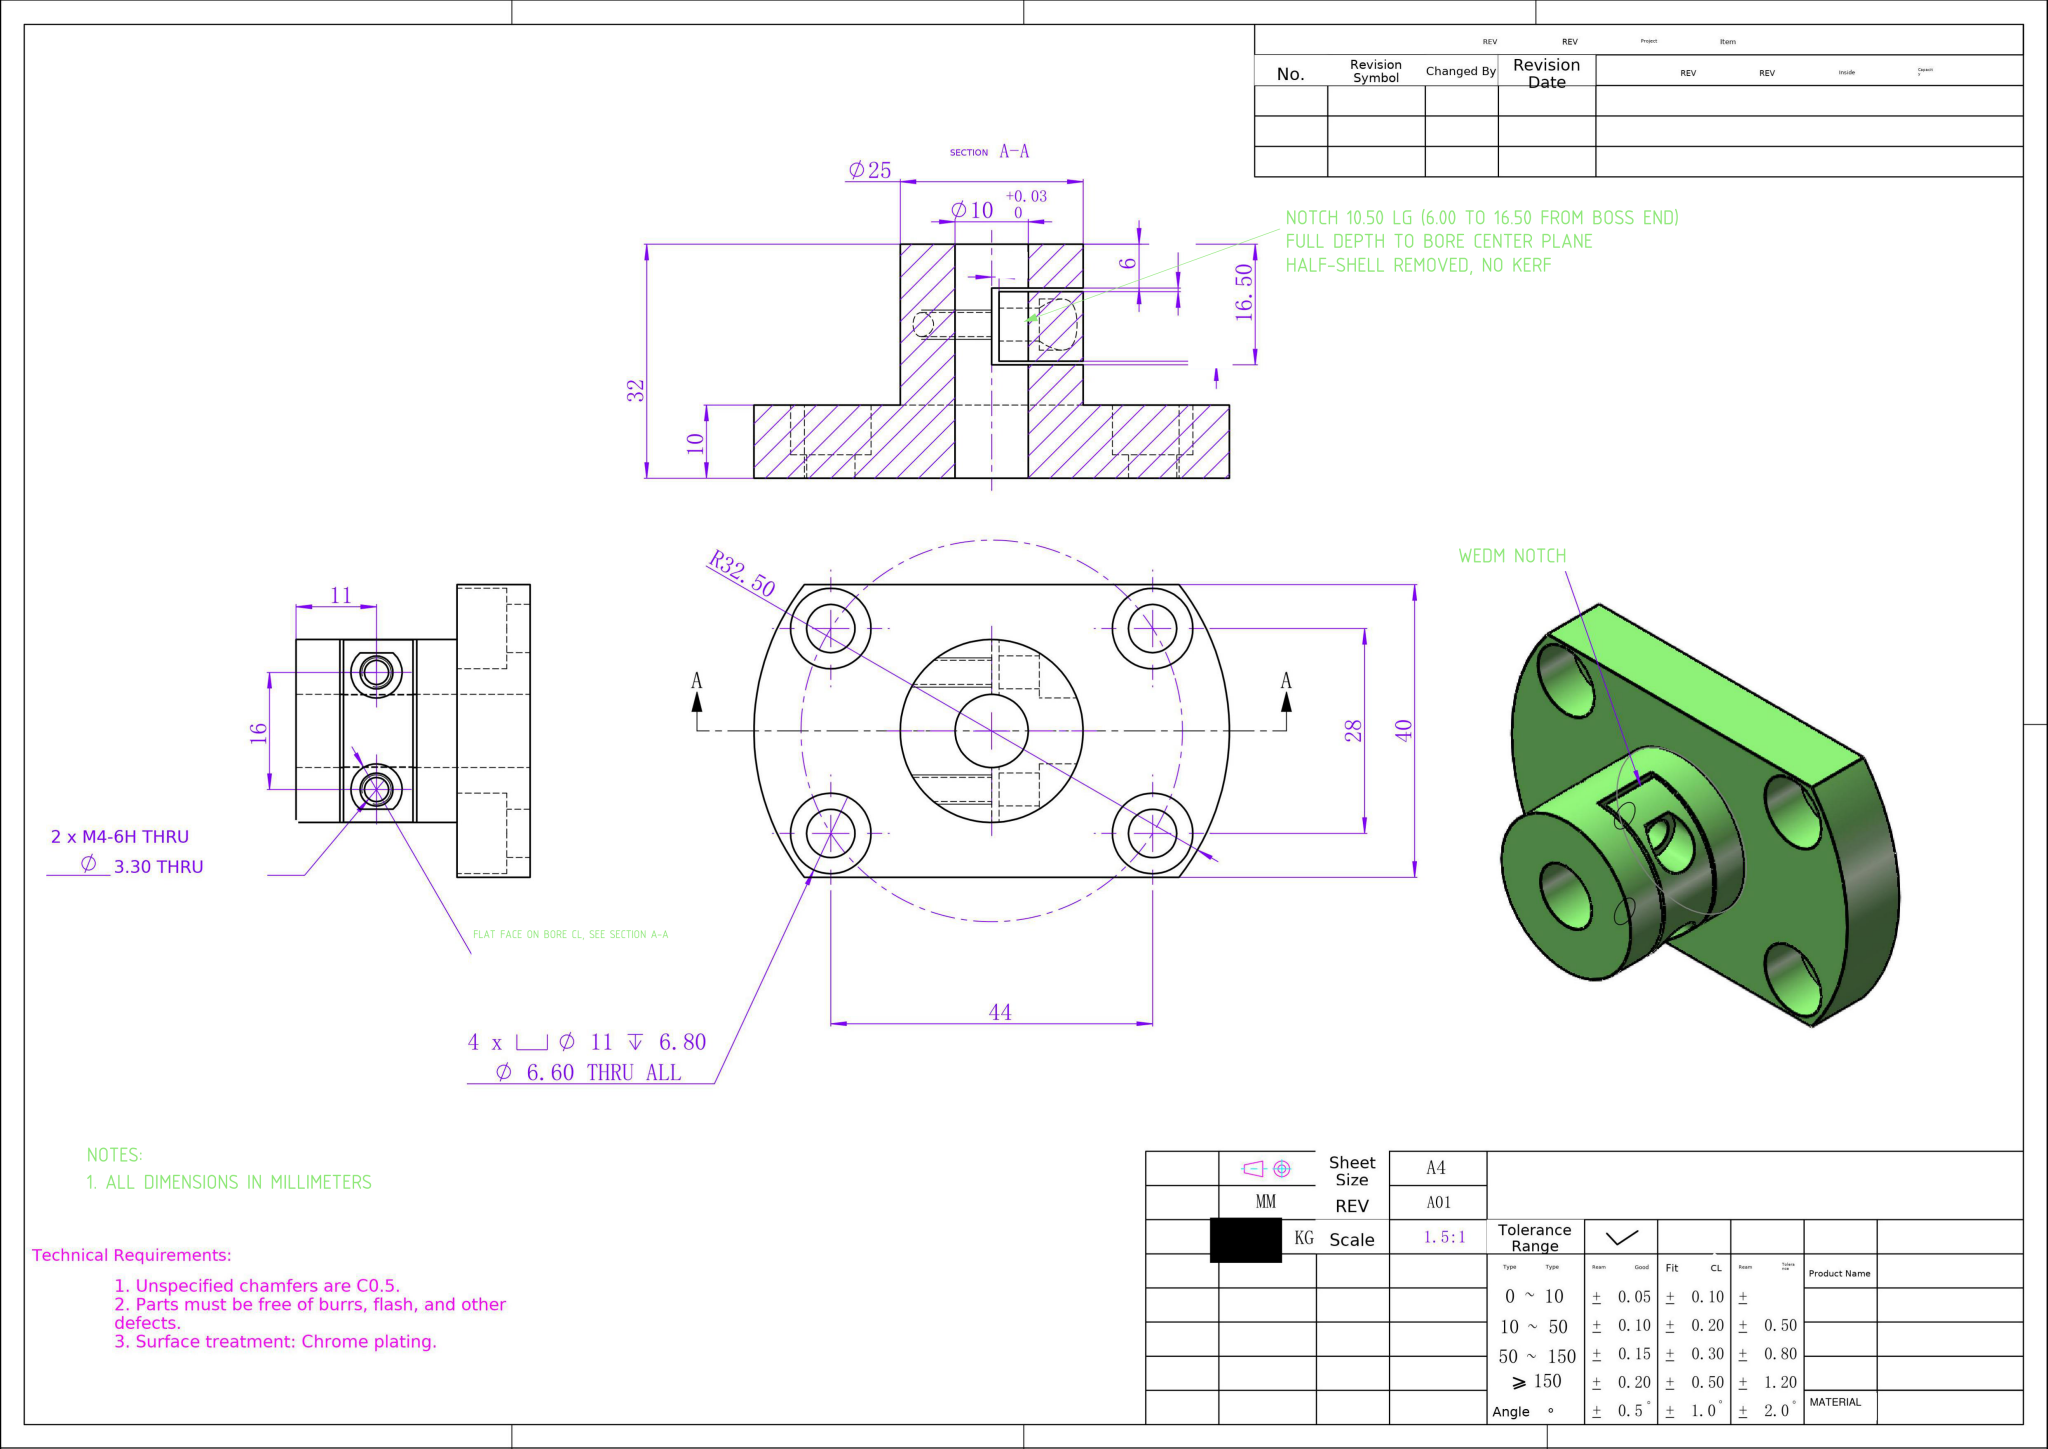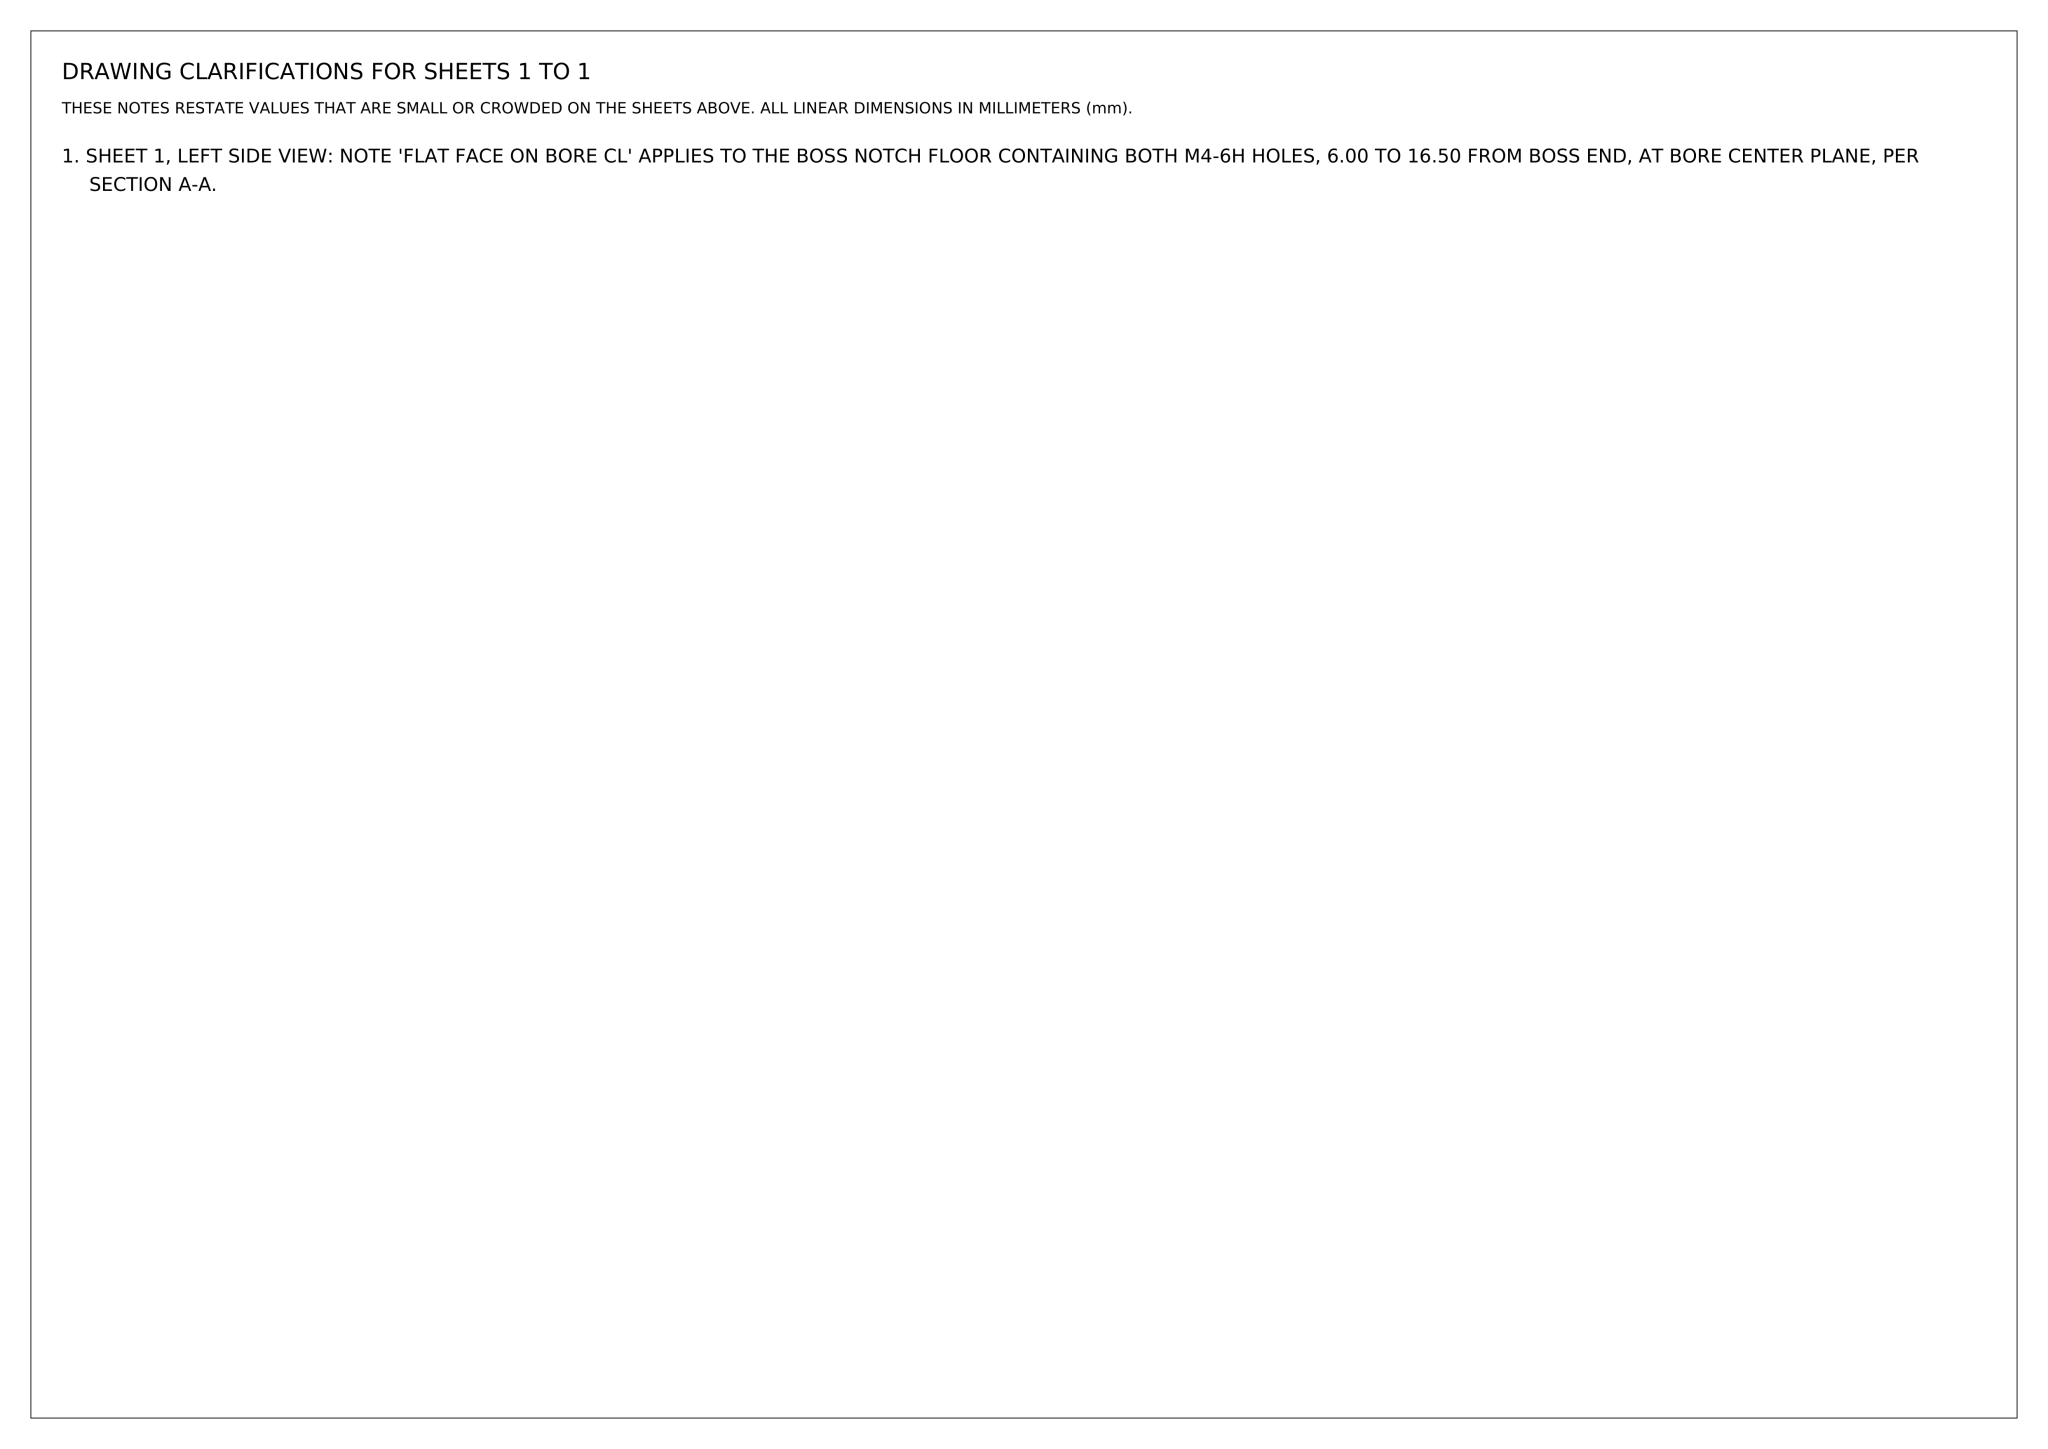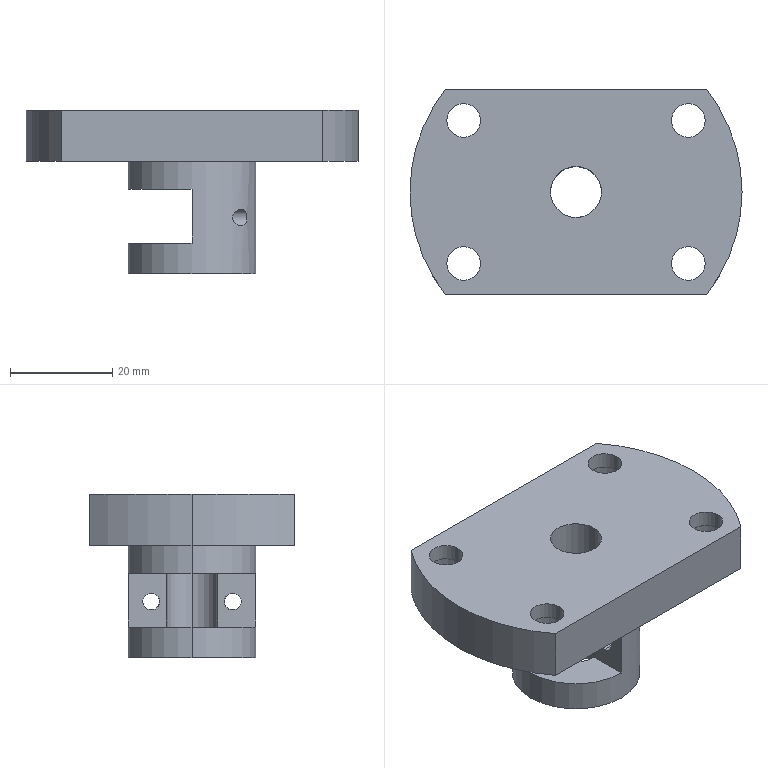Part | NX | mm | 1 solid | 40 faces | box 65 x 40 x 32 mm | volume 27186 mm3 | cylinder 27 | plane 13 | commonest cylinder face diameters 6.6 x8 11 x8 3.3 x4 65 x3 10 x2 25 x2